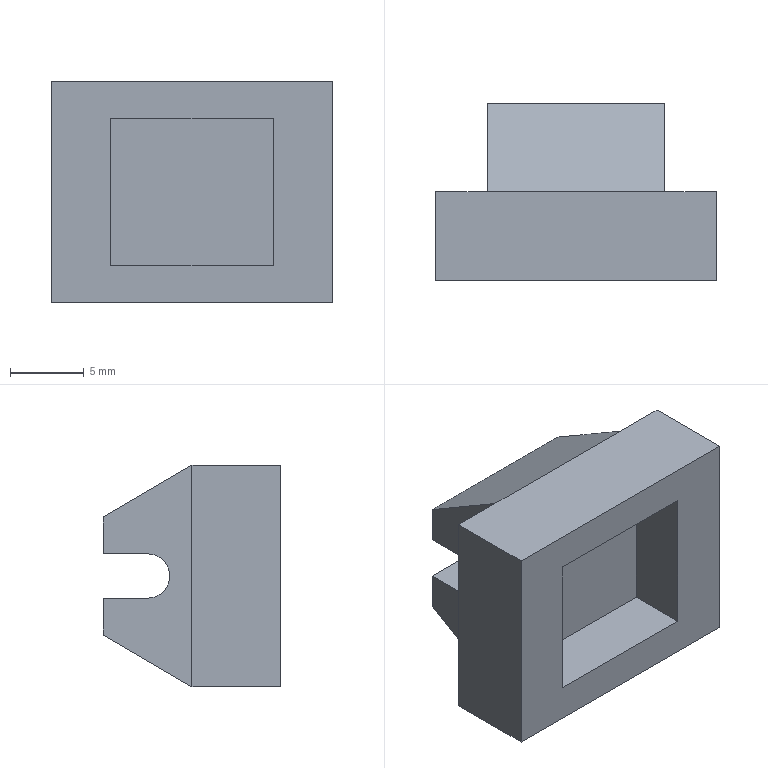Component | NX | LINK_6_SLIDER | 1 solid | 29 faces | volume 1771 mm3 | plane 27 | cylinder 2 | commonest cylinder face diameters 3 x2